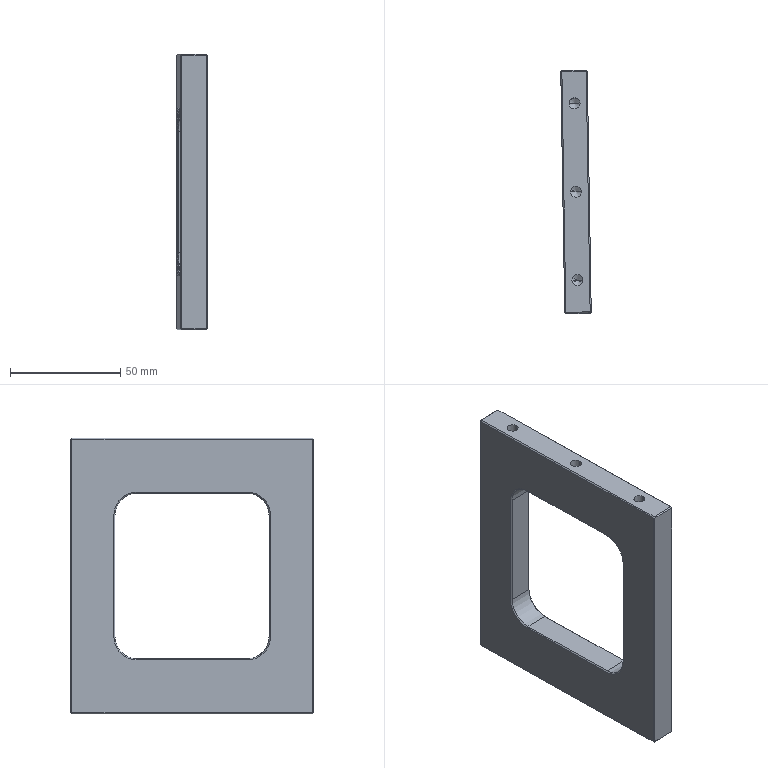Component | SolidWorks | 8TC-A17001-20-10MountingPlate2-3 | 1 solid | 74 faces | box 13.79 x 110.17 x 125 mm | volume 100777 mm3 | plane 38 | cone 20 | cylinder 16 | commonest cylinder face diameters 5 x12 20 x4 | material A3
build123d program:
from build123d import *

# Parameters (mm, degrees)
SKETCH1_W             = 110
SKETCH1_H             = 12
BOSS_EXTRUDE1_DEPTH   = 125
M6_TAPPED_HOLE1_D     = 5
M6_TAPPED_HOLE1_DEPTH = 17
M6_TAPPED_HOLE1_TIP   = 1.502
M6_TAPPED_HOLE2_D     = 5
M6_TAPPED_HOLE2_DEPTH = 17
M6_TAPPED_HOLE2_TIP   = 1.502
SKETCH6_W             = 70
SKETCH6_H             = 75
CUT_EXTRUDE1_DEPTH    = 138.091
FILLET1_R             = 10
CHAMFER1_SIZE         = 0.5


with BuildPart() as part:
    # Sketch1 → Boss-Extrude1 (new body)
    with BuildSketch(Plane(origin=(0, 0, 0), x_dir=(1, 0, 0), z_dir=(0, 1, 0))):
        Rectangle(SKETCH1_W, SKETCH1_H)
    extrude(amount=BOSS_EXTRUDE1_DEPTH)

    # M6 Tapped Hole1
    with Locations(Plane(origin=(0, 125, 0), x_dir=(1, 0, 0), z_dir=(0, 1, 0))):
        with Locations((40, 0), (0, 0), (-40, 0)):
            Hole(M6_TAPPED_HOLE1_D / 2, depth=M6_TAPPED_HOLE1_DEPTH)
            with Locations((0, 0, -(M6_TAPPED_HOLE1_DEPTH + M6_TAPPED_HOLE1_TIP / 2))):  # 118° drill point
                Cone(0, M6_TAPPED_HOLE1_D / 2, M6_TAPPED_HOLE1_TIP, mode=Mode.SUBTRACT)

    # M6 Tapped Hole2
    with Locations(Plane(origin=(0, 0, 0), x_dir=(-1, 0, 0), z_dir=(0, -1, 0))):
        with Locations((40, 0), (-40, 0), (0, 0)):
            Hole(M6_TAPPED_HOLE2_D / 2, depth=M6_TAPPED_HOLE2_DEPTH)
            with Locations((0, 0, -(M6_TAPPED_HOLE2_DEPTH + M6_TAPPED_HOLE2_TIP / 2))):  # 118° drill point
                Cone(0, M6_TAPPED_HOLE2_D / 2, M6_TAPPED_HOLE2_TIP, mode=Mode.SUBTRACT)

    # Sketch6 → Cut-Extrude1 (cut, through all)
    with BuildSketch(Plane.XY.offset(6)):
        with Locations((0, 62.5)):
            Rectangle(SKETCH6_W, SKETCH6_H)
    extrude(amount=-CUT_EXTRUDE1_DEPTH, mode=Mode.SUBTRACT)

    # Fillet1
    fillet1_edges = [part.edges().sort_by_distance(p)[0] for p in [
        (-35, 25, 0),
        (-35, 100, 0),
        (35, 100, 0),
        (35, 25, 0),
    ]]
    fillet(fillet1_edges, radius=FILLET1_R)

    # Chamfer1
    chamfer1_edges = [part.edges().sort_by_distance(p)[0] for p in [
        (-55, 125, 0),
        (0, 125, 6),
        (55, 125, 0),
        (0, 0, 6),
        (-55, 0, 0),
        (0, 0, -6),
        (35, 62.5, 6),
        (55, 0, 0),
        (35, 62.5, -6),
        (0, 25, 6),
        (0, 25, -6),
        (-35, 62.5, 6),
        (-35, 62.5, -6),
        (0, 100, 6),
        (0, 100, -6),
        (32.071, 27.929, 6),
        (32.071, 27.929, -6),
        (-32.071, 27.929, 6),
        (-32.071, 27.929, -6),
        (-32.071, 97.071, 6),
        (-32.071, 97.071, -6),
        (32.071, 97.071, 6),
        (32.071, 97.071, -6),
        (0, 125, -6),
        (55, 62.5, 6),
        (-55, 62.5, 6),
        (-55, 62.5, -6),
        (55, 62.5, -6),
    ]]
    chamfer(chamfer1_edges, length=CHAMFER1_SIZE)


solid = part.part

# Placed as in the assembly
solid = solid.moved(Location((671.537, 199.71, 30.814), (90, -89.057, 180)))